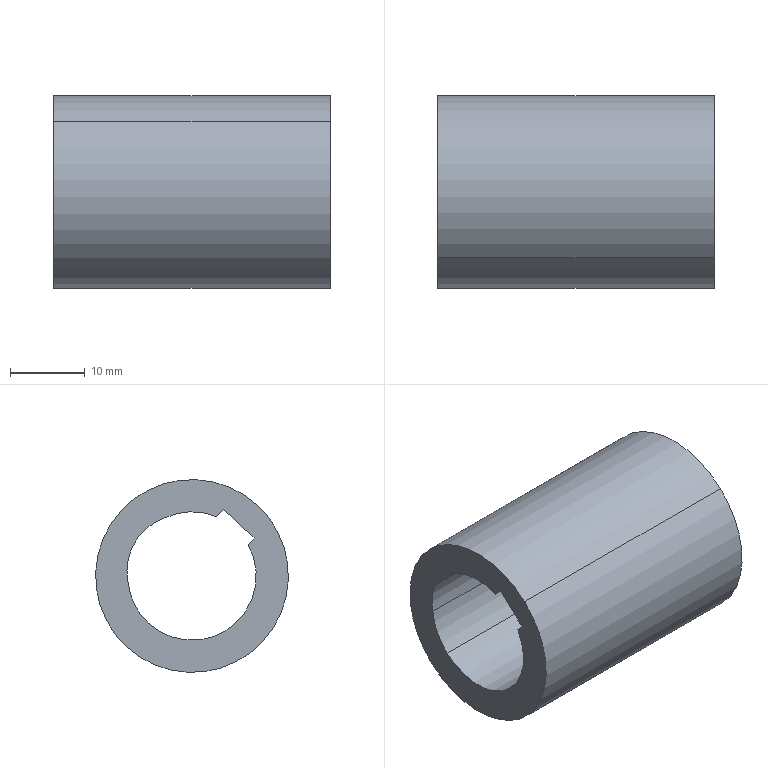Component | SolidWorks | CouplingSleeve-1 | 1 solid | 12 faces | box 37 x 25.76 x 25.76 mm | volume 10449 mm3 | cylinder 6 | plane 6 | commonest cylinder face diameters 17.16 x3 25.756 x2 15 x1
build123d program:
from build123d import *

# Parameters (mm, degrees)
SKETCH2_R                 = 12.878
SKETCH2_R_2               = 8.58
BOSS_EXTRUDE1_DEPTH       = 37
CUT_EXTRUDE1_2_DEPTH      = 66.986
CUT_EXTRUDE1_2_DEPTH_BACK = 66.986
CUT_EXTRUDE1_DEPTH        = 211.224
CUT_EXTRUDE1_DEPTH_BACK   = 211.224
SKETCH1_W                 = 4.594
SKETCH1_H                 = 0.62


with BuildPart() as part:
    # Sketch2 → Boss-Extrude1 (new body)
    with BuildSketch(Plane(origin=(-166, 0, 0), x_dir=(0, 0, -1), z_dir=(1, 0, 0))):
        with Locations((-40.219, 0)):
            Circle(SKETCH2_R)
        with Locations((-40.219, 0)):
            Circle(SKETCH2_R_2, mode=Mode.SUBTRACT)
    extrude(amount=-BOSS_EXTRUDE1_DEPTH)

    # Sketch4 → Cut-Extrude1_2 (cut, two sides: drawn at the far end of the back side and taken through both)
    with BuildSketch(Plane(origin=(-166, 0, 0), x_dir=(0, 0, -1), z_dir=(1, 0, 0)).offset(-CUT_EXTRUDE1_2_DEPTH_BACK)):
        with BuildLine():
            Line((-46.528, -2.177), (-49.594, -2.177))
            Line((-49.594, -2.177), (-49.594, 3.001))
            Line((-49.594, 3.001), (-47.204, 3.001))
            ThreePointArc((-47.204, 3.001), (-32.458, 2.295), (-46.528, -2.177))
        make_face()
    extrude(amount=CUT_EXTRUDE1_2_DEPTH + CUT_EXTRUDE1_2_DEPTH_BACK, mode=Mode.SUBTRACT)

    # Sketch1 → Cut-Extrude1 (cut, two sides: drawn at the far end of the back side and taken through both)
    with BuildSketch(Plane(origin=(0, 0, 0), x_dir=(0, 0, -1), z_dir=(1, 0, 0)).offset(-CUT_EXTRUDE1_DEPTH_BACK)):
        with Locations((-47.297, -2.31)):
            Rectangle(SKETCH1_W, SKETCH1_H)
    extrude(amount=CUT_EXTRUDE1_DEPTH + CUT_EXTRUDE1_DEPTH_BACK, mode=Mode.SUBTRACT)


solid = part.part

# Placed as in the assembly
solid = solid.moved(Location((-83.5, 87.608, -29.452), (42.922, 0, 0)))
STEP:
#1=CARTESIAN_POINT('',(-11.28,2.601,-0.2474));
#2=VERTEX_POINT('',#1);
#3=CARTESIAN_POINT('',(-11.28,2.707,-0.03261));
#4=VERTEX_POINT('',#3);
#5=CARTESIAN_POINT('',(-11.28,2.371,-0.));
#6=DIRECTION('',(1.,0.,0.));
#7=DIRECTION('',(0.,0.681,-0.7323));
#8=AXIS2_PLACEMENT_3D('',#5,#6,#7);
#9=CIRCLE('',#8,0.3378);
#10=EDGE_CURVE('',#2,#4,#9,.T.);
#11=ORIENTED_EDGE('',*,*,#10,.F.);
#12=CARTESIAN_POINT('',(-9.823,2.601,-0.2474));
#13=VERTEX_POINT('',#12);
#14=CARTESIAN_POINT('',(-11.28,2.601,-0.2474));
#15=DIRECTION('',(1.,0.,0.));
#16=VECTOR('',#15,39.37);
#17=LINE('',#14,#16);
#18=EDGE_CURVE('',#2,#13,#17,.T.);
#19=ORIENTED_EDGE('',*,*,#18,.T.);
#20=CARTESIAN_POINT('',(-9.823,2.707,-0.03261));
#21=VERTEX_POINT('',#20);
#22=CARTESIAN_POINT('',(-9.823,2.371,-0.));
#23=DIRECTION('',(1.,0.,0.));
#24=DIRECTION('',(0.,0.681,-0.7323));
#25=AXIS2_PLACEMENT_3D('',#22,#23,#24);
#26=CIRCLE('',#25,0.3378);
#27=EDGE_CURVE('',#13,#21,#26,.T.);
#28=ORIENTED_EDGE('',*,*,#27,.T.);
#29=CARTESIAN_POINT('',(-10.551,2.707,-0.03261));
#30=DIRECTION('',(-1.,0.,0.));
#31=VECTOR('',#30,39.37);
#32=LINE('',#29,#31);
#33=EDGE_CURVE('',#21,#4,#32,.T.);
#34=ORIENTED_EDGE('',*,*,#33,.T.);
#35=EDGE_LOOP('',(#11,#19,#28,#34));
#36=FACE_OUTER_BOUND('',#35,.T.);
#37=CARTESIAN_POINT('',(-11.28,2.371,-0.));
#38=DIRECTION('',(1.,0.,0.));
#39=DIRECTION('',(0.,0.681,-0.7323));
#40=AXIS2_PLACEMENT_3D('',#37,#38,#39);
#41=CYLINDRICAL_SURFACE('',#40,0.3378);
#42=ADVANCED_FACE('',(#36),#41,.F.);
#43=CARTESIAN_POINT('',(-11.28,2.716,-0.3713));
#44=VERTEX_POINT('',#43);
#45=CARTESIAN_POINT('',(-11.28,2.026,0.3713));
#46=VERTEX_POINT('',#45);
#47=CARTESIAN_POINT('',(-11.28,2.371,-0.));
#48=DIRECTION('',(1.,0.,0.));
#49=DIRECTION('',(0.,0.681,-0.7323));
#50=AXIS2_PLACEMENT_3D('',#47,#48,#49);
#51=CIRCLE('',#50,0.507);
#52=EDGE_CURVE('',#44,#46,#51,.T.);
#53=ORIENTED_EDGE('',*,*,#52,.T.);
#54=CARTESIAN_POINT('',(-9.823,2.026,0.3713));
#55=VERTEX_POINT('',#54);
#56=CARTESIAN_POINT('',(-11.28,2.026,0.3713));
#57=DIRECTION('',(1.,0.,0.));
#58=VECTOR('',#57,39.37);
#59=LINE('',#56,#58);
#60=EDGE_CURVE('',#46,#55,#59,.T.);
#61=ORIENTED_EDGE('',*,*,#60,.T.);
#62=CARTESIAN_POINT('',(-9.823,2.716,-0.3713));
#63=VERTEX_POINT('',#62);
#64=CARTESIAN_POINT('',(-9.823,2.371,-0.));
#65=DIRECTION('',(1.,0.,0.));
#66=DIRECTION('',(0.,0.681,-0.7323));
#67=AXIS2_PLACEMENT_3D('',#64,#65,#66);
#68=CIRCLE('',#67,0.507);
#69=EDGE_CURVE('',#63,#55,#68,.T.);
#70=ORIENTED_EDGE('',*,*,#69,.F.);
#71=CARTESIAN_POINT('',(-11.28,2.716,-0.3713));
#72=DIRECTION('',(1.,0.,0.));
#73=VECTOR('',#72,39.37);
#74=LINE('',#71,#73);
#75=EDGE_CURVE('',#44,#63,#74,.T.);
#76=ORIENTED_EDGE('',*,*,#75,.F.);
#77=EDGE_LOOP('',(#53,#61,#70,#76));
#78=FACE_OUTER_BOUND('',#77,.T.);
#79=CARTESIAN_POINT('',(-11.28,2.371,-0.));
#80=DIRECTION('',(1.,0.,0.));
#81=DIRECTION('',(0.,0.681,-0.7323));
#82=AXIS2_PLACEMENT_3D('',#79,#80,#81);
#83=CYLINDRICAL_SURFACE('',#82,0.507);
#84=ADVANCED_FACE('',(#78),#83,.T.);
#85=CARTESIAN_POINT('',(-11.28,2.52,0.3031));
#86=VERTEX_POINT('',#85);
#87=CARTESIAN_POINT('',(-11.28,2.242,0.3122));
#88=VERTEX_POINT('',#87);
#89=CARTESIAN_POINT('',(-11.28,2.371,-0.));
#90=DIRECTION('',(1.,0.,0.));
#91=DIRECTION('',(0.,0.681,-0.7323));
#92=AXIS2_PLACEMENT_3D('',#89,#90,#91);
#93=CIRCLE('',#92,0.3378);
#94=EDGE_CURVE('',#86,#88,#93,.T.);
#95=ORIENTED_EDGE('',*,*,#94,.F.);
#96=CARTESIAN_POINT('',(-9.823,2.52,0.3031));
#97=VERTEX_POINT('',#96);
#98=CARTESIAN_POINT('',(-10.551,2.52,0.3031));
#99=DIRECTION('',(1.,0.,0.));
#100=VECTOR('',#99,39.37);
#101=LINE('',#98,#100);
#102=EDGE_CURVE('',#86,#97,#101,.T.);
#103=ORIENTED_EDGE('',*,*,#102,.T.);
#104=CARTESIAN_POINT('',(-9.823,2.242,0.3122));
#105=VERTEX_POINT('',#104);
#106=CARTESIAN_POINT('',(-9.823,2.371,-0.));
#107=DIRECTION('',(1.,0.,0.));
#108=DIRECTION('',(0.,0.681,-0.7323));
#109=AXIS2_PLACEMENT_3D('',#106,#107,#108);
#110=CIRCLE('',#109,0.3378);
#111=EDGE_CURVE('',#97,#105,#110,.T.);
#112=ORIENTED_EDGE('',*,*,#111,.T.);
#113=CARTESIAN_POINT('',(-11.28,2.242,0.3122));
#114=DIRECTION('',(-1.,0.,0.));
#115=VECTOR('',#114,39.37);
#116=LINE('',#113,#115);
#117=EDGE_CURVE('',#105,#88,#116,.T.);
#118=ORIENTED_EDGE('',*,*,#117,.T.);
#119=EDGE_LOOP('',(#95,#103,#112,#118));
#120=FACE_OUTER_BOUND('',#119,.T.);
#121=CARTESIAN_POINT('',(-11.28,2.371,-0.));
#122=DIRECTION('',(1.,0.,0.));
#123=DIRECTION('',(0.,0.681,-0.7323));
#124=AXIS2_PLACEMENT_3D('',#121,#122,#123);
#125=CYLINDRICAL_SURFACE('',#124,0.3378);
#126=ADVANCED_FACE('',(#120),#125,.F.);
#127=ORIENTED_EDGE('',*,*,#60,.F.);
#128=CARTESIAN_POINT('',(-11.28,2.371,-0.));
#129=DIRECTION('',(1.,0.,0.));
#130=DIRECTION('',(0.,0.681,-0.7323));
#131=AXIS2_PLACEMENT_3D('',#128,#129,#130);
#132=CIRCLE('',#131,0.507);
#133=EDGE_CURVE('',#46,#44,#132,.T.);
#134=ORIENTED_EDGE('',*,*,#133,.T.);
#135=ORIENTED_EDGE('',*,*,#75,.T.);
#136=CARTESIAN_POINT('',(-9.823,2.371,-0.));
#137=DIRECTION('',(1.,0.,0.));
#138=DIRECTION('',(0.,0.681,-0.7323));
#139=AXIS2_PLACEMENT_3D('',#136,#137,#138);
#140=CIRCLE('',#139,0.507);
#141=EDGE_CURVE('',#55,#63,#140,.T.);
#142=ORIENTED_EDGE('',*,*,#141,.F.);
#143=EDGE_LOOP('',(#127,#134,#135,#142));
#144=FACE_OUTER_BOUND('',#143,.T.);
#145=CARTESIAN_POINT('',(-11.28,2.371,-0.));
#146=DIRECTION('',(1.,0.,0.));
#147=DIRECTION('',(0.,0.681,-0.7323));
#148=AXIS2_PLACEMENT_3D('',#145,#146,#147);
#149=CYLINDRICAL_SURFACE('',#148,0.507);
#150=ADVANCED_FACE('',(#144),#149,.T.);
#151=CARTESIAN_POINT('',(-11.28,2.057,0.2119));
#152=VERTEX_POINT('',#151);
#153=CARTESIAN_POINT('',(-11.28,2.044,0.2));
#154=VERTEX_POINT('',#153);
#155=CARTESIAN_POINT('',(-11.28,2.119,0.2703));
#156=DIRECTION('',(0.,-0.7323,-0.681));
#157=VECTOR('',#156,39.37);
#158=LINE('',#155,#157);
#159=EDGE_CURVE('',#152,#154,#158,.T.);
#160=ORIENTED_EDGE('',*,*,#159,.T.);
#161=CARTESIAN_POINT('',(-11.28,2.076,0.1653));
#162=VERTEX_POINT('',#161);
#163=CARTESIAN_POINT('',(-11.28,2.167,0.06759));
#164=DIRECTION('',(0.,0.681,-0.7323));
#165=VECTOR('',#164,39.37);
#166=LINE('',#163,#165);
#167=EDGE_CURVE('',#154,#162,#166,.T.);
#168=ORIENTED_EDGE('',*,*,#167,.T.);
#169=CARTESIAN_POINT('',(-11.28,2.371,-0.));
#170=DIRECTION('',(1.,0.,0.));
#171=DIRECTION('',(0.,0.681,-0.7323));
#172=AXIS2_PLACEMENT_3D('',#169,#170,#171);
#173=CIRCLE('',#172,0.3378);
#174=EDGE_CURVE('',#162,#2,#173,.T.);
#175=ORIENTED_EDGE('',*,*,#174,.T.);
#176=ORIENTED_EDGE('',*,*,#10,.T.);
#177=CARTESIAN_POINT('',(-11.28,2.418,0.02612));
#178=DIRECTION('',(1.,0.,0.));
#179=DIRECTION('',(0.,0.681,-0.7323));
#180=AXIS2_PLACEMENT_3D('',#177,#178,#179);
#181=CIRCLE('',#180,0.2953);
#182=EDGE_CURVE('',#4,#86,#181,.T.);
#183=ORIENTED_EDGE('',*,*,#182,.T.);
#184=ORIENTED_EDGE('',*,*,#94,.T.);
#185=CARTESIAN_POINT('',(-11.28,2.206,0.3507));
#186=VERTEX_POINT('',#185);
#187=CARTESIAN_POINT('',(-11.28,2.206,0.3507));
#188=DIRECTION('',(0.,-0.681,0.7323));
#189=VECTOR('',#188,39.37);
#190=LINE('',#187,#189);
#191=EDGE_CURVE('',#88,#186,#190,.T.);
#192=ORIENTED_EDGE('',*,*,#191,.T.);
#193=CARTESIAN_POINT('',(-11.28,2.119,0.2703));
#194=DIRECTION('',(0.,-0.7323,-0.681));
#195=VECTOR('',#194,39.37);
#196=LINE('',#193,#195);
#197=EDGE_CURVE('',#186,#152,#196,.T.);
#198=ORIENTED_EDGE('',*,*,#197,.T.);
#199=EDGE_LOOP('',(#160,#168,#175,#176,#183,#184,#192,#198));
#200=FACE_BOUND('',#199,.T.);
#201=ORIENTED_EDGE('',*,*,#52,.F.);
#202=ORIENTED_EDGE('',*,*,#133,.F.);
#203=EDGE_LOOP('',(#201,#202));
#204=FACE_OUTER_BOUND('',#203,.T.);
#205=CARTESIAN_POINT('',(-11.28,2.371,-0.));
#206=DIRECTION('',(1.,0.,0.));
#207=DIRECTION('',(0.,0.681,-0.7323));
#208=AXIS2_PLACEMENT_3D('',#205,#206,#207);
#209=PLANE('',#208);
#210=ADVANCED_FACE('',(#200,#204),#209,.F.);
#211=CARTESIAN_POINT('',(-9.823,2.044,0.2));
#212=VERTEX_POINT('',#211);
#213=CARTESIAN_POINT('',(-9.823,2.076,0.1653));
#214=VERTEX_POINT('',#213);
#215=CARTESIAN_POINT('',(-9.823,2.295,-0.07024));
#216=DIRECTION('',(0.,0.681,-0.7323));
#217=VECTOR('',#216,39.37);
#218=LINE('',#215,#217);
#219=EDGE_CURVE('',#212,#214,#218,.T.);
#220=ORIENTED_EDGE('',*,*,#219,.F.);
#221=CARTESIAN_POINT('',(-9.823,2.057,0.2119));
#222=VERTEX_POINT('',#221);
#223=CARTESIAN_POINT('',(-9.823,2.119,0.2703));
#224=DIRECTION('',(0.,-0.7323,-0.681));
#225=VECTOR('',#224,39.37);
#226=LINE('',#223,#225);
#227=EDGE_CURVE('',#222,#212,#226,.T.);
#228=ORIENTED_EDGE('',*,*,#227,.F.);
#229=CARTESIAN_POINT('',(-9.823,2.206,0.3507));
#230=VERTEX_POINT('',#229);
#231=CARTESIAN_POINT('',(-9.823,2.119,0.2703));
#232=DIRECTION('',(0.,-0.7323,-0.681));
#233=VECTOR('',#232,39.37);
#234=LINE('',#231,#233);
#235=EDGE_CURVE('',#230,#222,#234,.T.);
#236=ORIENTED_EDGE('',*,*,#235,.F.);
#237=CARTESIAN_POINT('',(-9.823,2.457,0.08045));
#238=DIRECTION('',(0.,-0.681,0.7323));
#239=VECTOR('',#238,39.37);
#240=LINE('',#237,#239);
#241=EDGE_CURVE('',#105,#230,#240,.T.);
#242=ORIENTED_EDGE('',*,*,#241,.F.);
#243=ORIENTED_EDGE('',*,*,#111,.F.);
#244=CARTESIAN_POINT('',(-9.823,2.418,0.02612));
#245=DIRECTION('',(1.,0.,0.));
#246=DIRECTION('',(0.,0.681,-0.7323));
#247=AXIS2_PLACEMENT_3D('',#244,#245,#246);
#248=CIRCLE('',#247,0.2953);
#249=EDGE_CURVE('',#21,#97,#248,.T.);
#250=ORIENTED_EDGE('',*,*,#249,.F.);
#251=ORIENTED_EDGE('',*,*,#27,.F.);
#252=CARTESIAN_POINT('',(-9.823,2.371,-0.));
#253=DIRECTION('',(1.,0.,0.));
#254=DIRECTION('',(0.,0.681,-0.7323));
#255=AXIS2_PLACEMENT_3D('',#252,#253,#254);
#256=CIRCLE('',#255,0.3378);
#257=EDGE_CURVE('',#214,#13,#256,.T.);
#258=ORIENTED_EDGE('',*,*,#257,.F.);
#259=EDGE_LOOP('',(#220,#228,#236,#242,#243,#250,#251,#258));
#260=FACE_BOUND('',#259,.T.);
#261=ORIENTED_EDGE('',*,*,#69,.T.);
#262=ORIENTED_EDGE('',*,*,#141,.T.);
#263=EDGE_LOOP('',(#261,#262));
#264=FACE_OUTER_BOUND('',#263,.T.);
#265=CARTESIAN_POINT('',(-9.823,2.371,-0.));
#266=DIRECTION('',(1.,0.,0.));
#267=DIRECTION('',(0.,0.681,-0.7323));
#268=AXIS2_PLACEMENT_3D('',#265,#266,#267);
#269=PLANE('',#268);
#270=ADVANCED_FACE('',(#260,#264),#269,.T.);
#271=ORIENTED_EDGE('',*,*,#18,.F.);
#272=ORIENTED_EDGE('',*,*,#174,.F.);
#273=CARTESIAN_POINT('',(-11.28,2.076,0.1653));
#274=DIRECTION('',(1.,0.,0.));
#275=VECTOR('',#274,39.37);
#276=LINE('',#273,#275);
#277=EDGE_CURVE('',#162,#214,#276,.T.);
#278=ORIENTED_EDGE('',*,*,#277,.T.);
#279=ORIENTED_EDGE('',*,*,#257,.T.);
#280=EDGE_LOOP('',(#271,#272,#278,#279));
#281=FACE_OUTER_BOUND('',#280,.T.);
#282=CARTESIAN_POINT('',(-11.28,2.371,-0.));
#283=DIRECTION('',(1.,0.,0.));
#284=DIRECTION('',(0.,0.681,-0.7323));
#285=AXIS2_PLACEMENT_3D('',#282,#283,#284);
#286=CYLINDRICAL_SURFACE('',#285,0.3378);
#287=ADVANCED_FACE('',(#281),#286,.F.);
#288=ORIENTED_EDGE('',*,*,#241,.T.);
#289=CARTESIAN_POINT('',(-11.28,2.206,0.3507));
#290=DIRECTION('',(1.,0.,0.));
#291=VECTOR('',#290,39.37);
#292=LINE('',#289,#291);
#293=EDGE_CURVE('',#186,#230,#292,.T.);
#294=ORIENTED_EDGE('',*,*,#293,.F.);
#295=ORIENTED_EDGE('',*,*,#191,.F.);
#296=ORIENTED_EDGE('',*,*,#117,.F.);
#297=EDGE_LOOP('',(#288,#294,#295,#296));
#298=FACE_OUTER_BOUND('',#297,.T.);
#299=CARTESIAN_POINT('',(-11.28,2.206,0.3507));
#300=DIRECTION('',(0.,0.7323,0.681));
#301=DIRECTION('',(0.,-0.681,0.7323));
#302=AXIS2_PLACEMENT_3D('',#299,#300,#301);
#303=PLANE('',#302);
#304=ADVANCED_FACE('',(#298),#303,.F.);
#305=CARTESIAN_POINT('',(-11.28,2.057,0.2119));
#306=CARTESIAN_POINT('',(-10.794,2.057,0.2119));
#307=CARTESIAN_POINT('',(-10.308,2.057,0.2119));
#308=CARTESIAN_POINT('',(-9.823,2.057,0.2119));
#309=B_SPLINE_CURVE_WITH_KNOTS('',3,(#305,#306,#307,#308),.UNSPECIFIED.,.F.,.F.,(4,4),(0.,1.),.UNSPECIFIED.);
#310=EDGE_CURVE('',#152,#222,#309,.T.);
#311=ORIENTED_EDGE('',*,*,#310,.F.);
#312=ORIENTED_EDGE('',*,*,#197,.F.);
#313=ORIENTED_EDGE('',*,*,#293,.T.);
#314=ORIENTED_EDGE('',*,*,#235,.T.);
#315=EDGE_LOOP('',(#311,#312,#313,#314));
#316=FACE_OUTER_BOUND('',#315,.T.);
#317=CARTESIAN_POINT('',(-11.28,2.057,0.2119));
#318=DIRECTION('',(0.,-0.681,0.7323));
#319=DIRECTION('',(1.,0.,0.));
#320=AXIS2_PLACEMENT_3D('',#317,#318,#319);
#321=PLANE('',#320);
#322=ADVANCED_FACE('',(#316),#321,.F.);
#323=ORIENTED_EDGE('',*,*,#182,.F.);
#324=ORIENTED_EDGE('',*,*,#33,.F.);
#325=ORIENTED_EDGE('',*,*,#249,.T.);
#326=ORIENTED_EDGE('',*,*,#102,.F.);
#327=EDGE_LOOP('',(#323,#324,#325,#326));
#328=FACE_OUTER_BOUND('',#327,.T.);
#329=CARTESIAN_POINT('',(-11.28,2.418,0.02612));
#330=DIRECTION('',(1.,0.,0.));
#331=DIRECTION('',(0.,0.681,-0.7323));
#332=AXIS2_PLACEMENT_3D('',#329,#330,#331);
#333=CYLINDRICAL_SURFACE('',#332,0.2953);
#334=ADVANCED_FACE('',(#328),#333,.F.);
#335=ORIENTED_EDGE('',*,*,#219,.T.);
#336=ORIENTED_EDGE('',*,*,#277,.F.);
#337=ORIENTED_EDGE('',*,*,#167,.F.);
#338=CARTESIAN_POINT('',(-11.28,2.044,0.2));
#339=DIRECTION('',(1.,0.,0.));
#340=VECTOR('',#339,39.37);
#341=LINE('',#338,#340);
#342=EDGE_CURVE('',#154,#212,#341,.T.);
#343=ORIENTED_EDGE('',*,*,#342,.T.);
#344=EDGE_LOOP('',(#335,#336,#337,#343));
#345=FACE_OUTER_BOUND('',#344,.T.);
#346=CARTESIAN_POINT('',(-11.28,2.167,0.06759));
#347=DIRECTION('',(0.,-0.7323,-0.681));
#348=DIRECTION('',(0.,0.681,-0.7323));
#349=AXIS2_PLACEMENT_3D('',#346,#347,#348);
#350=PLANE('',#349);
#351=ADVANCED_FACE('',(#345),#350,.F.);
#352=ORIENTED_EDGE('',*,*,#310,.T.);
#353=ORIENTED_EDGE('',*,*,#227,.T.);
#354=ORIENTED_EDGE('',*,*,#342,.F.);
#355=ORIENTED_EDGE('',*,*,#159,.F.);
#356=EDGE_LOOP('',(#352,#353,#354,#355));
#357=FACE_OUTER_BOUND('',#356,.T.);
#358=CARTESIAN_POINT('',(-11.28,2.044,0.2));
#359=DIRECTION('',(0.,-0.681,0.7323));
#360=DIRECTION('',(1.,0.,0.));
#361=AXIS2_PLACEMENT_3D('',#358,#359,#360);
#362=PLANE('',#361);
#363=ADVANCED_FACE('',(#357),#362,.F.);
#364=CLOSED_SHELL('',(#42,#84,#126,#150,#210,#270,#287,#304,#322,#334,#351,#363));
#365=MANIFOLD_SOLID_BREP('',#364);
#366=CARTESIAN_POINT('',(0.,0.,0.));
#367=DIRECTION('',(0.,0.,1.));
#368=DIRECTION('',(1.,0.,0.));
#369=AXIS2_PLACEMENT_3D('',#366,#367,#368);
#370=(LENGTH_UNIT()NAMED_UNIT(*)SI_UNIT($,.METRE.));
#371=LENGTH_MEASURE_WITH_UNIT(LENGTH_MEASURE(0.0254),#370);
#372=DIMENSIONAL_EXPONENTS(1.,0.,0.,0.,0.,0.,0.);
#373=(CONVERSION_BASED_UNIT('',#371)LENGTH_UNIT()NAMED_UNIT(#372));
#374=UNCERTAINTY_MEASURE_WITH_UNIT(LENGTH_MEASURE(0.00001),#373,'','');
#375=(NAMED_UNIT(*)PLANE_ANGLE_UNIT()SI_UNIT($,.RADIAN.));
#376=(NAMED_UNIT(*)SI_UNIT($,.STERADIAN.)SOLID_ANGLE_UNIT());
#377=(GEOMETRIC_REPRESENTATION_CONTEXT(3)GLOBAL_UNCERTAINTY_ASSIGNED_CONTEXT((#374))GLOBAL_UNIT_ASSIGNED_CONTEXT((#373,#375,#376))REPRESENTATION_CONTEXT('',''));
#378=ADVANCED_BREP_SHAPE_REPRESENTATION('',(#365,#369),#377);
#379=COLOUR_RGB('',0.7922,0.8196,0.9333);
#380=FILL_AREA_STYLE_COLOUR('',#379);
#381=FILL_AREA_STYLE('',(#380));
#382=SURFACE_STYLE_FILL_AREA(#381);
#383=SURFACE_SIDE_STYLE('',(#382));
#384=SURFACE_STYLE_USAGE(.BOTH.,#383);
#385=PRESENTATION_STYLE_ASSIGNMENT((#384));
#386=STYLED_ITEM('',(#385),#365);
#387=(LENGTH_UNIT()NAMED_UNIT(*)SI_UNIT($,.METRE.));
#388=LENGTH_MEASURE_WITH_UNIT(LENGTH_MEASURE(0.0254),#387);
#389=DIMENSIONAL_EXPONENTS(1.,0.,0.,0.,0.,0.,0.);
#390=(CONVERSION_BASED_UNIT('',#388)LENGTH_UNIT()NAMED_UNIT(#389));
#391=UNCERTAINTY_MEASURE_WITH_UNIT(LENGTH_MEASURE(0.00001),#390,'','');
#392=(NAMED_UNIT(*)PLANE_ANGLE_UNIT()SI_UNIT($,.RADIAN.));
#393=(NAMED_UNIT(*)SI_UNIT($,.STERADIAN.)SOLID_ANGLE_UNIT());
#394=(GEOMETRIC_REPRESENTATION_CONTEXT(3)GLOBAL_UNCERTAINTY_ASSIGNED_CONTEXT((#391))GLOBAL_UNIT_ASSIGNED_CONTEXT((#390,#392,#393))REPRESENTATION_CONTEXT('',''));
#395=MECHANICAL_DESIGN_GEOMETRIC_PRESENTATION_REPRESENTATION('',(#386),#394);
#396=PRESENTATION_LAYER_ASSIGNMENT('','',(#386));